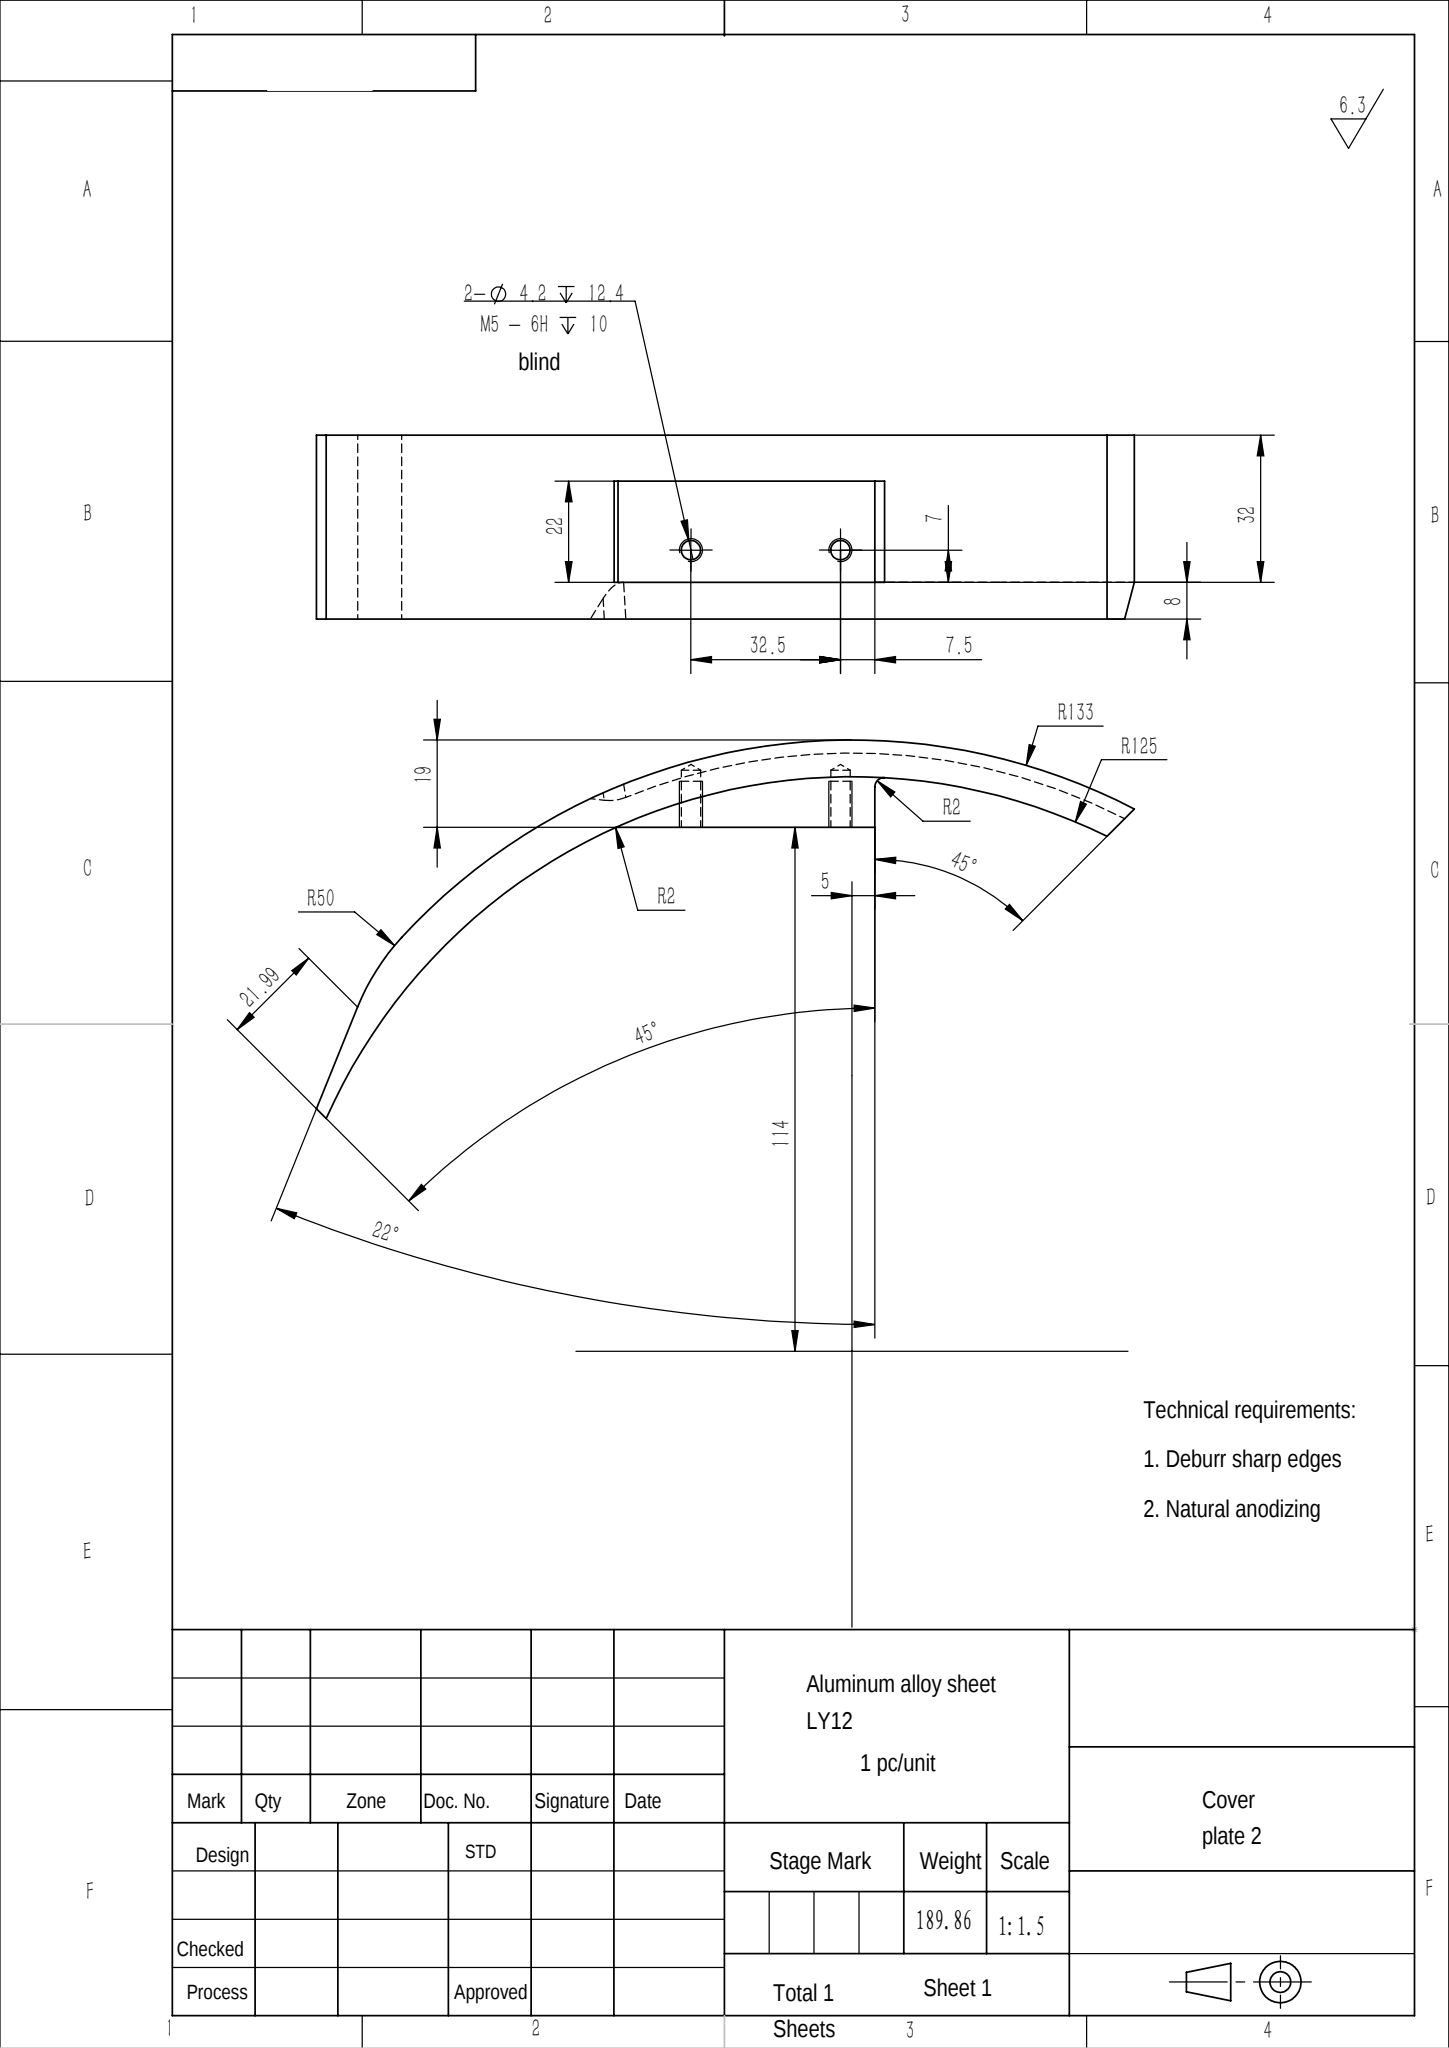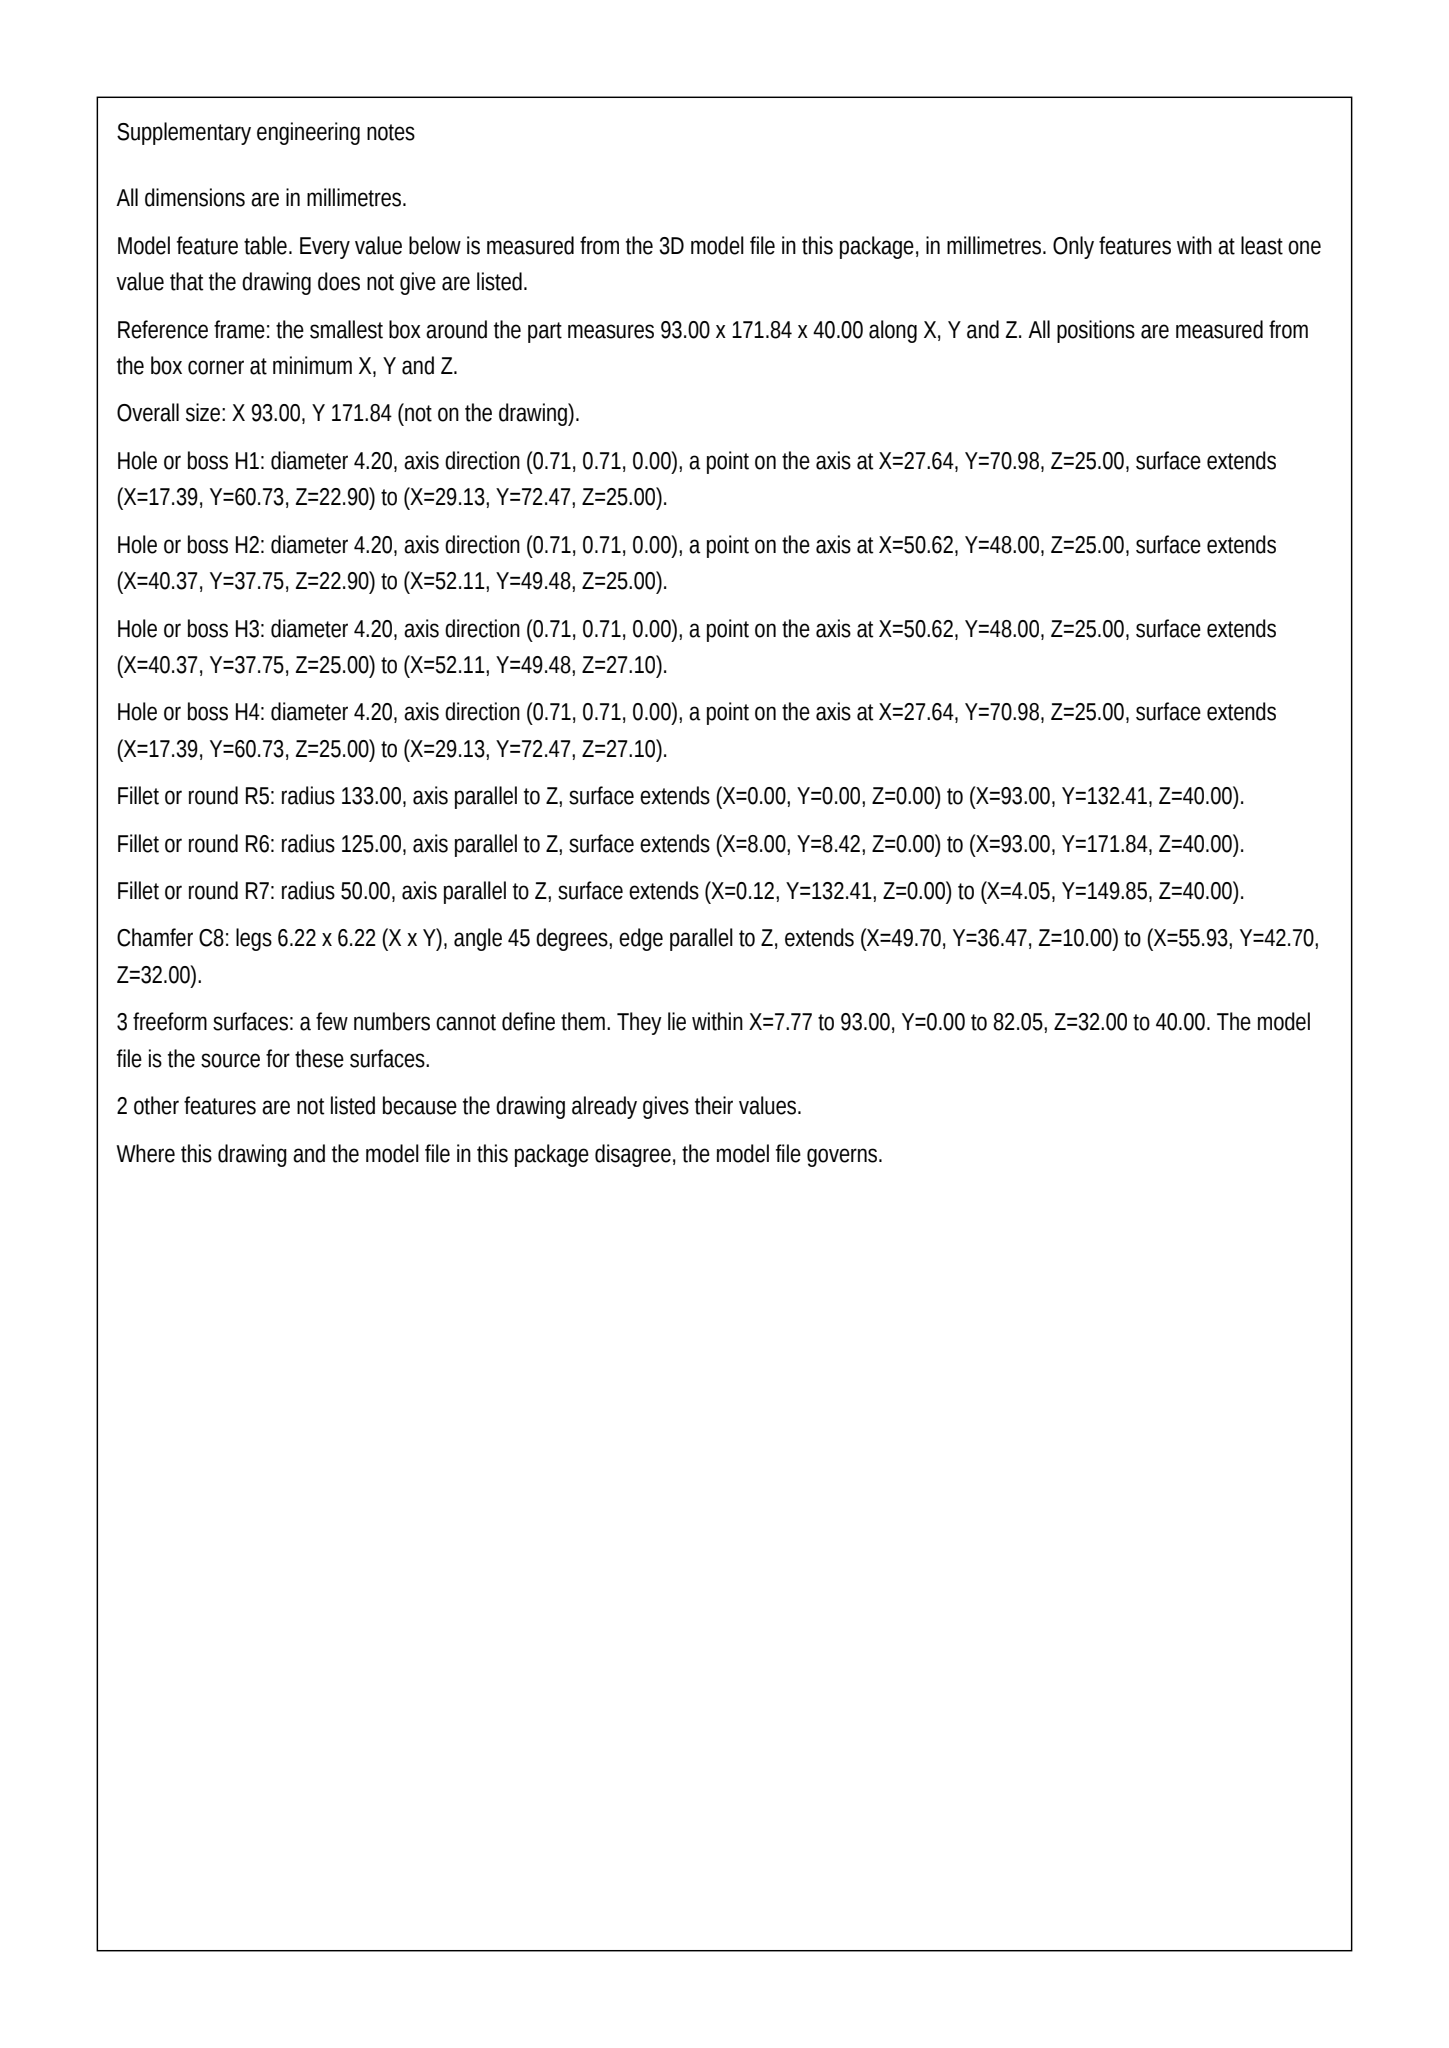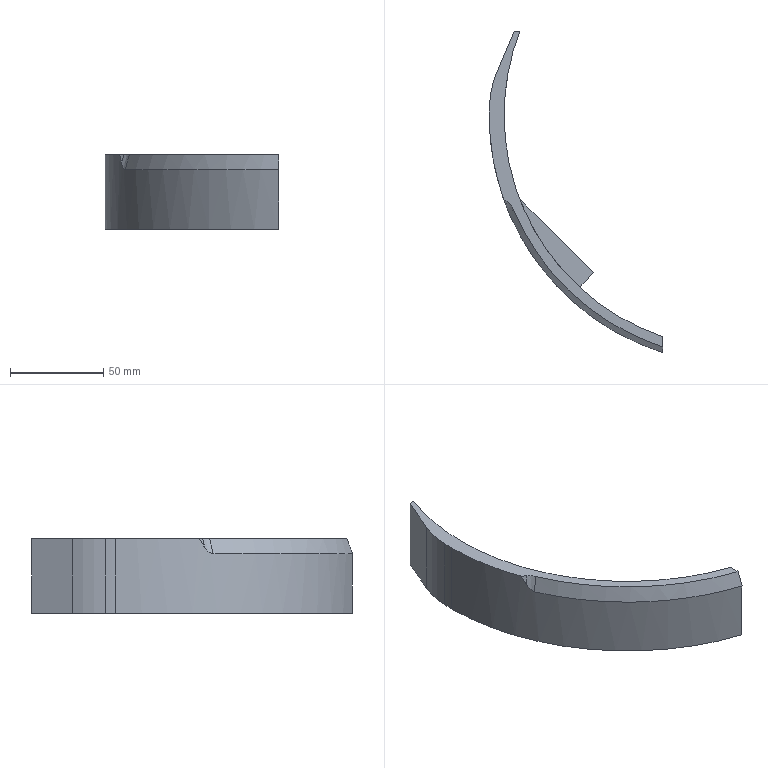Part | SolidWorks | mm | material Aluminum alloy sheet LY12 | 1 solid | 28 faces | box 93 x 171.84 x 40 mm | volume 70321 mm3 | cylinder 12 | plane 9 | cone 4 | spline 3 | commonest cylinder face diameters 4.2 x4 4 x3 266 x2 250 x2 100 x1